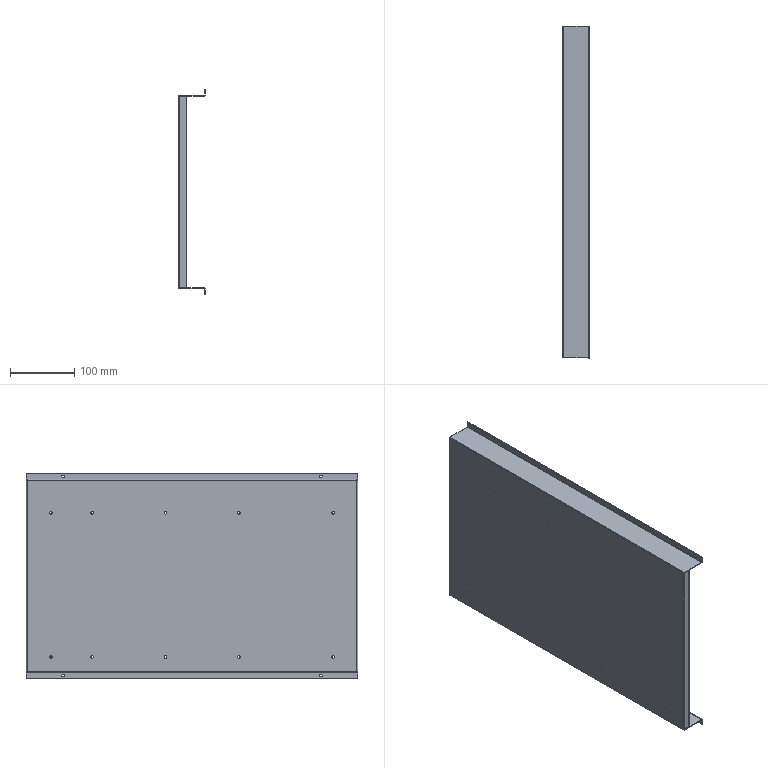Component | SolidWorks | PC-CAJ-P08-1_PM-CAJ-P62-1 | 1 solid | 86 faces | volume 210680 mm3 | plane 46 | cylinder 40 | commonest cylinder face diameters 4 x28 3 x6 1 x6 | material Plain Carbon Steel